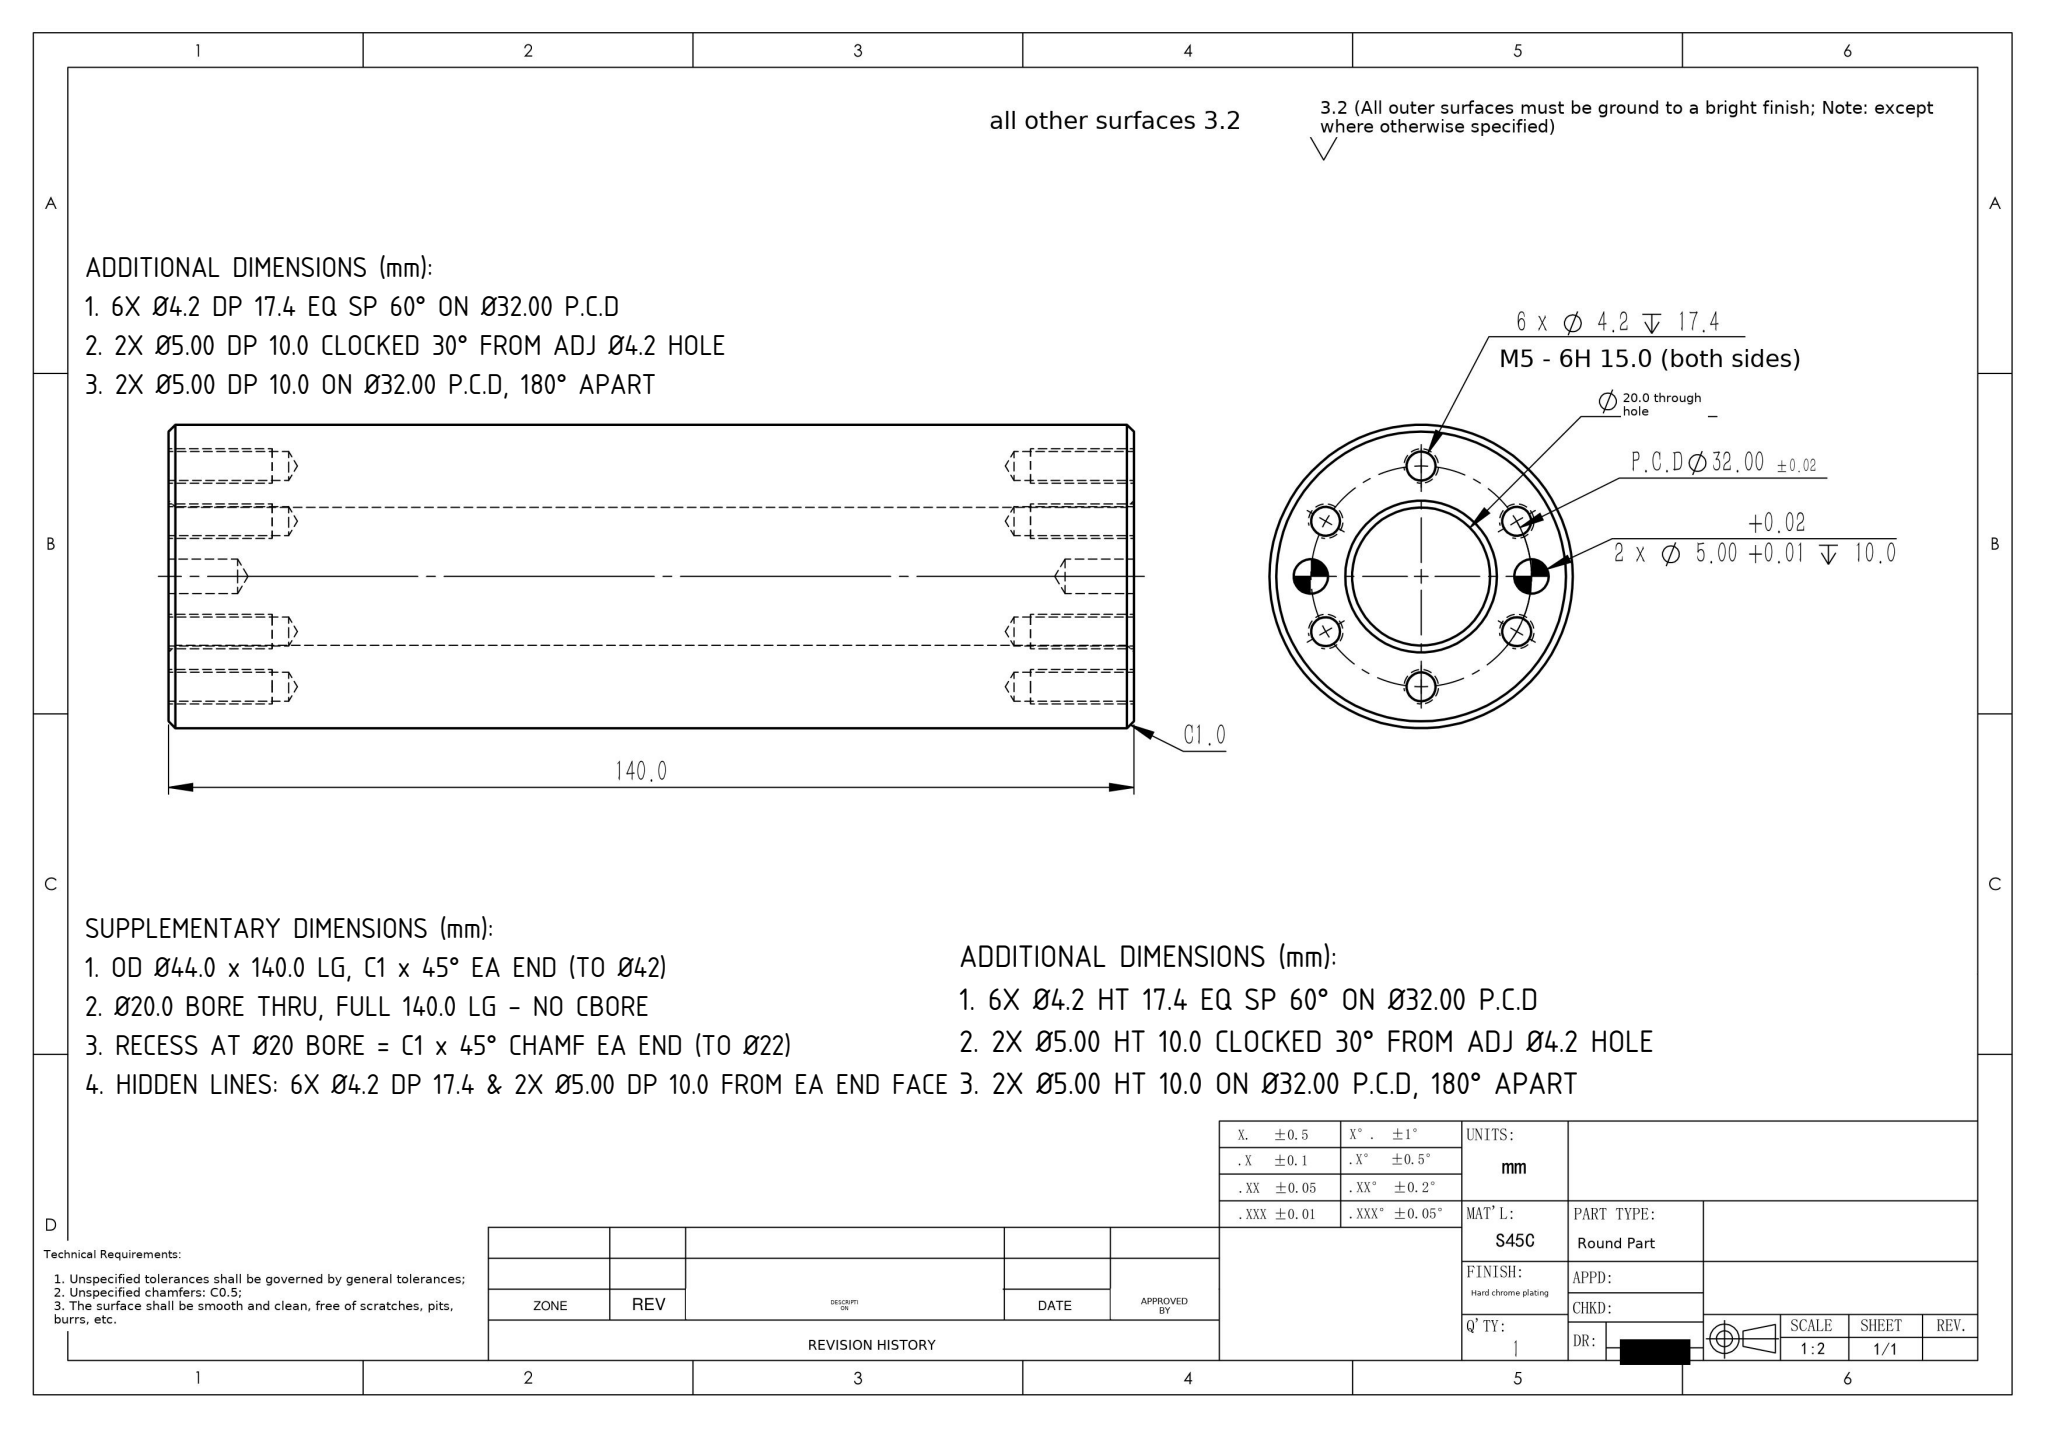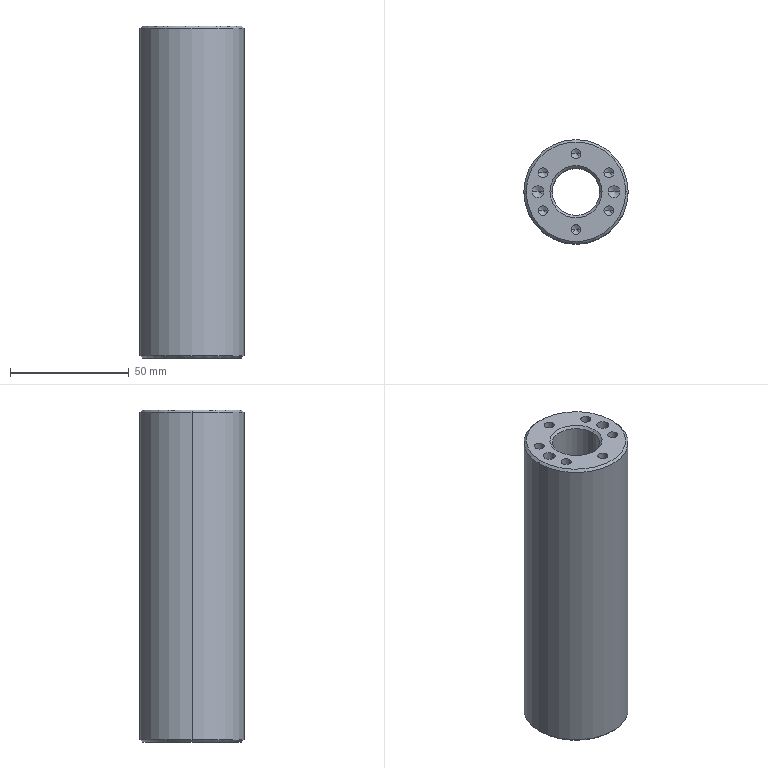Part | SolidWorks | mm | 1 solid | 78 faces | box 44 x 44 x 140 mm | volume 164904 mm3 | cone 40 | cylinder 36 | plane 2 | commonest cylinder face diameters 4.2 x24 5 x8 20 x2 44 x2
build123d program:
from build123d import *

# Parameters (mm, degrees)
SKETCH1_R                     = 22
SKETCH1_R_2                   = 10
BOSS_EXTRUDE1_DEPTH           = 140
CIRPATTERN1_COUNT             = 6
SIZE_MM_DOWEL_PIN_HOLE1_D     = 5
SIZE_MM_DOWEL_PIN_HOLE1_DEPTH = 10
SIZE_MM_DOWEL_PIN_HOLE1_TIP   = 1.502
SIZE_MM_DOWEL_PIN_HOLE2_D     = 5
SIZE_MM_DOWEL_PIN_HOLE2_DEPTH = 10
SIZE_MM_DOWEL_PIN_HOLE2_TIP   = 1.502
CHAMFER1_SIZE                 = 1


with BuildPart() as part:
    # Sketch1 → Boss-Extrude1 (new body)
    with BuildSketch(Plane.XY):
        Circle(SKETCH1_R)
        Circle(SKETCH1_R_2, mode=Mode.SUBTRACT)
    extrude(amount=BOSS_EXTRUDE1_DEPTH)

    # Sketch3 → M5 Tapped Hole1 (revolve, cut)
    with BuildSketch(Plane(origin=(0, 16, 0), x_dir=(0, 1, 0), z_dir=(1, 0, 0))):
        Polygon((0, 0), (0, 18.662), (2.1, 17.4), (2.1, 0), align=None)
    m5_tapped_hole1 = revolve(axis=Axis((0, 16, -6.35), (0, 0, 1)), mode=Mode.SUBTRACT)

    # Sketch5 → M5 Tapped Hole2 (revolve, cut)
    with BuildSketch(Plane(origin=(0, 16, 140), x_dir=(0, -1, 0), z_dir=(1, 0, 0))):
        Polygon((0, 0), (0, 18.662), (2.1, 17.4), (2.1, 0), align=None)
    m5_tapped_hole2 = revolve(axis=Axis((0, 16, 146.35), (0, 0, -1)), mode=Mode.SUBTRACT)

    # CirPattern1: M5 Tapped Hole1, M5 Tapped Hole2 ×6 about axis
    cirpattern1_axis = Axis((0, 0, 0), (0, 0, 1))
    add([m5_tapped_hole1.rotate(cirpattern1_axis, i * 360 / CIRPATTERN1_COUNT) for i in range(1, CIRPATTERN1_COUNT)], mode=Mode.SUBTRACT)
    add([m5_tapped_hole2.rotate(cirpattern1_axis, i * 360 / CIRPATTERN1_COUNT) for i in range(1, CIRPATTERN1_COUNT)], mode=Mode.SUBTRACT)

    # Size mm Dowel Pin Hole1
    with Locations(Plane.XY.offset(140)):
        with Locations((-16, 0), (16, 0)):
            Hole(SIZE_MM_DOWEL_PIN_HOLE1_D / 2, depth=SIZE_MM_DOWEL_PIN_HOLE1_DEPTH)
            with Locations((0, 0, -(SIZE_MM_DOWEL_PIN_HOLE1_DEPTH + SIZE_MM_DOWEL_PIN_HOLE1_TIP / 2))):  # 118° drill point
                Cone(0, SIZE_MM_DOWEL_PIN_HOLE1_D / 2, SIZE_MM_DOWEL_PIN_HOLE1_TIP, mode=Mode.SUBTRACT)

    # Size mm Dowel Pin Hole2
    with Locations(Plane(origin=(0, 0, 0), x_dir=(-1, 0, 0), z_dir=(0, 0, -1))):
        with Locations((-16, 0), (16, 0)):
            Hole(SIZE_MM_DOWEL_PIN_HOLE2_D / 2, depth=SIZE_MM_DOWEL_PIN_HOLE2_DEPTH)
            with Locations((0, 0, -(SIZE_MM_DOWEL_PIN_HOLE2_DEPTH + SIZE_MM_DOWEL_PIN_HOLE2_TIP / 2))):  # 118° drill point
                Cone(0, SIZE_MM_DOWEL_PIN_HOLE2_D / 2, SIZE_MM_DOWEL_PIN_HOLE2_TIP, mode=Mode.SUBTRACT)

    # Chamfer1
    chamfer1_edges = [part.edges().sort_by_distance(p)[0] for p in [
        (-22, 0, 0),
        (-22, 0, 140),
        (-10, 0, 0),
        (-10, 0, 140),
    ]]
    chamfer(chamfer1_edges, length=CHAMFER1_SIZE)


solid = part.part